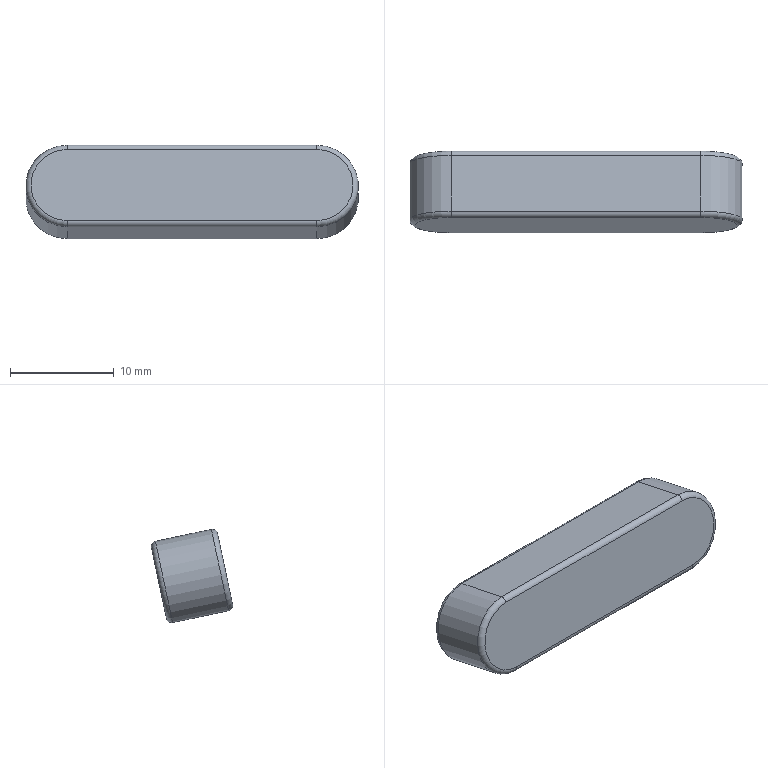Component | SolidWorks | 28ParallelKey8X32-1 | 1 solid | 14 faces | box 32 x 7.84 x 8.99 mm | volume 1567 mm3 | cylinder 6 | plane 4 | torus 4 | commonest cylinder face diameters 1 x4 8 x2
build123d program:
from build123d import *

# Parameters (mm, degrees)
BOSS_EXTRUDE1_DEPTH = 6.5
FILLET1_R           = 0.5


with BuildPart() as part:
    # Sketch1 → Boss-Extrude1 (new body)
    with BuildSketch(Plane(origin=(0, 0, 0), x_dir=(1, 0, 0), z_dir=(0, 1, 0))):
        with BuildLine():
            Line((-12, 4), (12, 4))
            ThreePointArc((12, 4), (16, 0), (12, -4))
            Line((12, -4), (-12, -4))
            ThreePointArc((-12, -4), (-16, 0), (-12, 4))
        make_face()
    extrude(amount=BOSS_EXTRUDE1_DEPTH)

    # Fillet1
    fillet1_edges = [part.edges().sort_by_distance(p)[0] for p in [
        (16, 6.5, 0),
        (0, 6.5, -4),
        (-16, 6.5, 0),
        (0, 0, -4),
        (16, 0, 0),
        (0, 0, 4),
        (-16, 0, 0),
        (0, 6.5, 4),
    ]]
    fillet(fillet1_edges, radius=FILLET1_R)


solid = part.part

# Placed as in the assembly
solid = solid.moved(Location((22.957, -20.232, 254.678), (168, 0, 0)))
STEP:
#1=COLOUR_RGB('',0.7922,0.8196,0.9333);
#2=FILL_AREA_STYLE_COLOUR('',#1);
#3=FILL_AREA_STYLE('',(#2));
#4=SURFACE_STYLE_FILL_AREA(#3);
#5=SURFACE_SIDE_STYLE('',(#4));
#6=SURFACE_STYLE_USAGE(.BOTH.,#5);
#7=PRESENTATION_STYLE_ASSIGNMENT((#6));
#8=CARTESIAN_POINT('',(0.4314,-0.8485,9.877));
#9=VERTEX_POINT('',#8);
#10=CARTESIAN_POINT('',(0.4314,-1.06,9.922));
#11=VERTEX_POINT('',#10);
#12=CARTESIAN_POINT('',(0.4314,-0.8293,9.873));
#13=DIRECTION('',(-0.,-0.9781,0.2079));
#14=VECTOR('',#13,39.37);
#15=LINE('',#12,#14);
#16=EDGE_CURVE('',#9,#11,#15,.T.);
#17=ORIENTED_EDGE('',*,*,#16,.T.);
#18=CARTESIAN_POINT('',(0.4314,-0.9949,10.23));
#19=VERTEX_POINT('',#18);
#20=CARTESIAN_POINT('',(0.4314,-1.028,10.076));
#21=DIRECTION('',(0.,0.9781,-0.2079));
#22=DIRECTION('',(0.,0.2079,0.9781));
#23=AXIS2_PLACEMENT_3D('',#20,#21,#22);
#24=CIRCLE('',#23,0.1575);
#25=EDGE_CURVE('',#11,#19,#24,.T.);
#26=ORIENTED_EDGE('',*,*,#25,.T.);
#27=CARTESIAN_POINT('',(0.4314,-0.7831,10.185));
#28=VERTEX_POINT('',#27);
#29=CARTESIAN_POINT('',(0.4314,-0.7638,10.181));
#30=DIRECTION('',(-0.,-0.9781,0.2079));
#31=VECTOR('',#30,39.37);
#32=LINE('',#29,#31);
#33=EDGE_CURVE('',#28,#19,#32,.T.);
#34=ORIENTED_EDGE('',*,*,#33,.F.);
#35=CARTESIAN_POINT('',(0.4314,-0.8158,10.031));
#36=DIRECTION('',(-0.,-0.9781,0.2079));
#37=DIRECTION('',(0.,0.2079,0.9781));
#38=AXIS2_PLACEMENT_3D('',#35,#36,#37);
#39=CIRCLE('',#38,0.1575);
#40=EDGE_CURVE('',#28,#9,#39,.T.);
#41=ORIENTED_EDGE('',*,*,#40,.T.);
#42=EDGE_LOOP('',(#17,#26,#34,#41));
#43=FACE_OUTER_BOUND('',#42,.T.);
#44=CARTESIAN_POINT('',(0.4314,-0.7965,10.027));
#45=DIRECTION('',(-0.,-0.9781,0.2079));
#46=DIRECTION('',(0.,-0.2079,-0.9781));
#47=AXIS2_PLACEMENT_3D('',#44,#45,#46);
#48=CYLINDRICAL_SURFACE('',#47,0.1575);
#49=ADVANCED_FACE('',(#43),#48,.T.);
#50=ORIENTED_EDGE('',*,*,#33,.T.);
#51=CARTESIAN_POINT('',(1.376,-0.9949,10.23));
#52=VERTEX_POINT('',#51);
#53=CARTESIAN_POINT('',(0.4314,-0.9949,10.23));
#54=DIRECTION('',(1.,-0.,0.));
#55=VECTOR('',#54,39.37);
#56=LINE('',#53,#55);
#57=EDGE_CURVE('',#19,#52,#56,.T.);
#58=ORIENTED_EDGE('',*,*,#57,.T.);
#59=CARTESIAN_POINT('',(1.376,-0.7831,10.185));
#60=VERTEX_POINT('',#59);
#61=CARTESIAN_POINT('',(1.376,-0.7638,10.181));
#62=DIRECTION('',(-0.,-0.9781,0.2079));
#63=VECTOR('',#62,39.37);
#64=LINE('',#61,#63);
#65=EDGE_CURVE('',#60,#52,#64,.T.);
#66=ORIENTED_EDGE('',*,*,#65,.F.);
#67=CARTESIAN_POINT('',(0.4314,-0.7831,10.185));
#68=DIRECTION('',(-1.,0.,-0.));
#69=VECTOR('',#68,39.37);
#70=LINE('',#67,#69);
#71=EDGE_CURVE('',#60,#28,#70,.T.);
#72=ORIENTED_EDGE('',*,*,#71,.T.);
#73=EDGE_LOOP('',(#50,#58,#66,#72));
#74=FACE_OUTER_BOUND('',#73,.T.);
#75=CARTESIAN_POINT('',(0.4314,-0.7638,10.181));
#76=DIRECTION('',(0.,-0.2079,-0.9781));
#77=DIRECTION('',(-1.,0.,-0.));
#78=AXIS2_PLACEMENT_3D('',#75,#76,#77);
#79=PLANE('',#78);
#80=ADVANCED_FACE('',(#74),#79,.F.);
#81=ORIENTED_EDGE('',*,*,#65,.T.);
#82=CARTESIAN_POINT('',(1.376,-1.06,9.922));
#83=VERTEX_POINT('',#82);
#84=CARTESIAN_POINT('',(1.376,-1.028,10.076));
#85=DIRECTION('',(0.,0.9781,-0.2079));
#86=DIRECTION('',(0.,0.2079,0.9781));
#87=AXIS2_PLACEMENT_3D('',#84,#85,#86);
#88=CIRCLE('',#87,0.1575);
#89=EDGE_CURVE('',#52,#83,#88,.T.);
#90=ORIENTED_EDGE('',*,*,#89,.T.);
#91=CARTESIAN_POINT('',(1.376,-0.8485,9.877));
#92=VERTEX_POINT('',#91);
#93=CARTESIAN_POINT('',(1.376,-0.8293,9.873));
#94=DIRECTION('',(-0.,-0.9781,0.2079));
#95=VECTOR('',#94,39.37);
#96=LINE('',#93,#95);
#97=EDGE_CURVE('',#92,#83,#96,.T.);
#98=ORIENTED_EDGE('',*,*,#97,.F.);
#99=CARTESIAN_POINT('',(1.376,-0.8158,10.031));
#100=DIRECTION('',(-0.,-0.9781,0.2079));
#101=DIRECTION('',(0.,0.2079,0.9781));
#102=AXIS2_PLACEMENT_3D('',#99,#100,#101);
#103=CIRCLE('',#102,0.1575);
#104=EDGE_CURVE('',#92,#60,#103,.T.);
#105=ORIENTED_EDGE('',*,*,#104,.T.);
#106=EDGE_LOOP('',(#81,#90,#98,#105));
#107=FACE_OUTER_BOUND('',#106,.T.);
#108=CARTESIAN_POINT('',(1.376,-0.7965,10.027));
#109=DIRECTION('',(-0.,-0.9781,0.2079));
#110=DIRECTION('',(0.,-0.2079,-0.9781));
#111=AXIS2_PLACEMENT_3D('',#108,#109,#110);
#112=CYLINDRICAL_SURFACE('',#111,0.1575);
#113=ADVANCED_FACE('',(#107),#112,.T.);
#114=ORIENTED_EDGE('',*,*,#97,.T.);
#115=CARTESIAN_POINT('',(0.4314,-1.06,9.922));
#116=DIRECTION('',(-1.,0.,-0.));
#117=VECTOR('',#116,39.37);
#118=LINE('',#115,#117);
#119=EDGE_CURVE('',#83,#11,#118,.T.);
#120=ORIENTED_EDGE('',*,*,#119,.T.);
#121=ORIENTED_EDGE('',*,*,#16,.F.);
#122=CARTESIAN_POINT('',(1.376,-0.8485,9.877));
#123=DIRECTION('',(1.,-0.,0.));
#124=VECTOR('',#123,39.37);
#125=LINE('',#122,#124);
#126=EDGE_CURVE('',#9,#92,#125,.T.);
#127=ORIENTED_EDGE('',*,*,#126,.T.);
#128=EDGE_LOOP('',(#114,#120,#121,#127));
#129=FACE_OUTER_BOUND('',#128,.T.);
#130=CARTESIAN_POINT('',(0.4314,-0.8293,9.873));
#131=DIRECTION('',(-0.,0.2079,0.9781));
#132=DIRECTION('',(1.,-0.,0.));
#133=AXIS2_PLACEMENT_3D('',#130,#131,#132);
#134=PLANE('',#133);
#135=ADVANCED_FACE('',(#129),#134,.F.);
#136=CARTESIAN_POINT('',(1.376,-0.7679,10.161));
#137=VERTEX_POINT('',#136);
#138=CARTESIAN_POINT('',(1.376,-0.8252,9.892));
#139=VERTEX_POINT('',#138);
#140=CARTESIAN_POINT('',(1.376,-0.7965,10.027));
#141=DIRECTION('',(0.,0.9781,-0.2079));
#142=DIRECTION('',(0.,0.2079,0.9781));
#143=AXIS2_PLACEMENT_3D('',#140,#141,#142);
#144=CIRCLE('',#143,0.1378);
#145=EDGE_CURVE('',#137,#139,#144,.T.);
#146=ORIENTED_EDGE('',*,*,#145,.T.);
#147=CARTESIAN_POINT('',(0.4314,-0.8252,9.892));
#148=VERTEX_POINT('',#147);
#149=CARTESIAN_POINT('',(0.4314,-0.8252,9.892));
#150=DIRECTION('',(-1.,0.,-0.));
#151=VECTOR('',#150,39.37);
#152=LINE('',#149,#151);
#153=EDGE_CURVE('',#139,#148,#152,.T.);
#154=ORIENTED_EDGE('',*,*,#153,.T.);
#155=CARTESIAN_POINT('',(0.4314,-0.7679,10.161));
#156=VERTEX_POINT('',#155);
#157=CARTESIAN_POINT('',(0.4314,-0.7965,10.027));
#158=DIRECTION('',(0.,0.9781,-0.2079));
#159=DIRECTION('',(0.,0.2079,0.9781));
#160=AXIS2_PLACEMENT_3D('',#157,#158,#159);
#161=CIRCLE('',#160,0.1378);
#162=EDGE_CURVE('',#148,#156,#161,.T.);
#163=ORIENTED_EDGE('',*,*,#162,.T.);
#164=CARTESIAN_POINT('',(1.376,-0.7679,10.161));
#165=DIRECTION('',(1.,-0.,0.));
#166=VECTOR('',#165,39.37);
#167=LINE('',#164,#166);
#168=EDGE_CURVE('',#156,#137,#167,.T.);
#169=ORIENTED_EDGE('',*,*,#168,.T.);
#170=EDGE_LOOP('',(#146,#154,#163,#169));
#171=FACE_OUTER_BOUND('',#170,.T.);
#172=CARTESIAN_POINT('',(0.4314,-0.7965,10.027));
#173=DIRECTION('',(0.,0.9781,-0.2079));
#174=DIRECTION('',(-0.,0.2079,0.9781));
#175=AXIS2_PLACEMENT_3D('',#172,#173,#174);
#176=PLANE('',#175);
#177=ADVANCED_FACE('',(#171),#176,.T.);
#178=CARTESIAN_POINT('',(1.376,-1.076,9.945));
#179=VERTEX_POINT('',#178);
#180=CARTESIAN_POINT('',(1.376,-1.018,10.215));
#181=VERTEX_POINT('',#180);
#182=CARTESIAN_POINT('',(1.376,-1.047,10.08));
#183=DIRECTION('',(-0.,-0.9781,0.2079));
#184=DIRECTION('',(0.,0.2079,0.9781));
#185=AXIS2_PLACEMENT_3D('',#182,#183,#184);
#186=CIRCLE('',#185,0.1378);
#187=EDGE_CURVE('',#179,#181,#186,.T.);
#188=ORIENTED_EDGE('',*,*,#187,.T.);
#189=CARTESIAN_POINT('',(0.4314,-1.018,10.215));
#190=VERTEX_POINT('',#189);
#191=CARTESIAN_POINT('',(0.4314,-1.018,10.215));
#192=DIRECTION('',(-1.,0.,-0.));
#193=VECTOR('',#192,39.37);
#194=LINE('',#191,#193);
#195=EDGE_CURVE('',#181,#190,#194,.T.);
#196=ORIENTED_EDGE('',*,*,#195,.T.);
#197=CARTESIAN_POINT('',(0.4314,-1.076,9.945));
#198=VERTEX_POINT('',#197);
#199=CARTESIAN_POINT('',(0.4314,-1.047,10.08));
#200=DIRECTION('',(-0.,-0.9781,0.2079));
#201=DIRECTION('',(0.,0.2079,0.9781));
#202=AXIS2_PLACEMENT_3D('',#199,#200,#201);
#203=CIRCLE('',#202,0.1378);
#204=EDGE_CURVE('',#190,#198,#203,.T.);
#205=ORIENTED_EDGE('',*,*,#204,.T.);
#206=CARTESIAN_POINT('',(0.4314,-1.076,9.945));
#207=DIRECTION('',(1.,-0.,0.));
#208=VECTOR('',#207,39.37);
#209=LINE('',#206,#208);
#210=EDGE_CURVE('',#198,#179,#209,.T.);
#211=ORIENTED_EDGE('',*,*,#210,.T.);
#212=EDGE_LOOP('',(#188,#196,#205,#211));
#213=FACE_OUTER_BOUND('',#212,.T.);
#214=CARTESIAN_POINT('',(0.4314,-1.047,10.08));
#215=DIRECTION('',(0.,0.9781,-0.2079));
#216=DIRECTION('',(-0.,0.2079,0.9781));
#217=AXIS2_PLACEMENT_3D('',#214,#215,#216);
#218=PLANE('',#217);
#219=ADVANCED_FACE('',(#213),#218,.F.);
#220=CARTESIAN_POINT('',(1.376,-1.056,9.941));
#221=DIRECTION('',(1.,-0.,0.));
#222=DIRECTION('',(0.,-0.2079,-0.9781));
#223=AXIS2_PLACEMENT_3D('',#220,#221,#222);
#224=CIRCLE('',#223,0.01969);
#225=EDGE_CURVE('',#179,#83,#224,.T.);
#226=ORIENTED_EDGE('',*,*,#225,.F.);
#227=ORIENTED_EDGE('',*,*,#210,.F.);
#228=CARTESIAN_POINT('',(0.4314,-1.056,9.941));
#229=DIRECTION('',(-1.,0.,-0.));
#230=DIRECTION('',(0.,0.2079,0.9781));
#231=AXIS2_PLACEMENT_3D('',#228,#229,#230);
#232=CIRCLE('',#231,0.01969);
#233=EDGE_CURVE('',#11,#198,#232,.T.);
#234=ORIENTED_EDGE('',*,*,#233,.F.);
#235=ORIENTED_EDGE('',*,*,#119,.F.);
#236=EDGE_LOOP('',(#226,#227,#234,#235));
#237=FACE_OUTER_BOUND('',#236,.T.);
#238=CARTESIAN_POINT('',(0.4314,-1.056,9.941));
#239=DIRECTION('',(-1.,0.,-0.));
#240=DIRECTION('',(0.,0.2079,0.9781));
#241=AXIS2_PLACEMENT_3D('',#238,#239,#240);
#242=CYLINDRICAL_SURFACE('',#241,0.01969);
#243=ADVANCED_FACE('',(#237),#242,.T.);
#244=ORIENTED_EDGE('',*,*,#233,.T.);
#245=ORIENTED_EDGE('',*,*,#204,.F.);
#246=CARTESIAN_POINT('',(0.4314,-0.999,10.211));
#247=DIRECTION('',(1.,-0.,0.));
#248=DIRECTION('',(0.,-0.2079,-0.9781));
#249=AXIS2_PLACEMENT_3D('',#246,#247,#248);
#250=CIRCLE('',#249,0.01969);
#251=EDGE_CURVE('',#19,#190,#250,.T.);
#252=ORIENTED_EDGE('',*,*,#251,.F.);
#253=ORIENTED_EDGE('',*,*,#25,.F.);
#254=EDGE_LOOP('',(#244,#245,#252,#253));
#255=FACE_OUTER_BOUND('',#254,.T.);
#256=CARTESIAN_POINT('',(0.4314,-1.028,10.076));
#257=DIRECTION('',(0.,0.9781,-0.2079));
#258=DIRECTION('',(0.,0.2079,0.9781));
#259=AXIS2_PLACEMENT_3D('',#256,#257,#258);
#260=TOROIDAL_SURFACE('',#259,0.1378,0.01969);
#261=ADVANCED_FACE('',(#255),#260,.T.);
#262=ORIENTED_EDGE('',*,*,#225,.T.);
#263=ORIENTED_EDGE('',*,*,#89,.F.);
#264=CARTESIAN_POINT('',(1.376,-0.999,10.211));
#265=DIRECTION('',(-1.,0.,-0.));
#266=DIRECTION('',(0.,0.2079,0.9781));
#267=AXIS2_PLACEMENT_3D('',#264,#265,#266);
#268=CIRCLE('',#267,0.01969);
#269=EDGE_CURVE('',#181,#52,#268,.T.);
#270=ORIENTED_EDGE('',*,*,#269,.F.);
#271=ORIENTED_EDGE('',*,*,#187,.F.);
#272=EDGE_LOOP('',(#262,#263,#270,#271));
#273=FACE_OUTER_BOUND('',#272,.T.);
#274=CARTESIAN_POINT('',(1.376,-1.028,10.076));
#275=DIRECTION('',(0.,0.9781,-0.2079));
#276=DIRECTION('',(0.,0.2079,0.9781));
#277=AXIS2_PLACEMENT_3D('',#274,#275,#276);
#278=TOROIDAL_SURFACE('',#277,0.1378,0.01969);
#279=ADVANCED_FACE('',(#273),#278,.T.);
#280=ORIENTED_EDGE('',*,*,#251,.T.);
#281=ORIENTED_EDGE('',*,*,#195,.F.);
#282=ORIENTED_EDGE('',*,*,#269,.T.);
#283=ORIENTED_EDGE('',*,*,#57,.F.);
#284=EDGE_LOOP('',(#280,#281,#282,#283));
#285=FACE_OUTER_BOUND('',#284,.T.);
#286=CARTESIAN_POINT('',(0.4314,-0.999,10.211));
#287=DIRECTION('',(1.,-0.,0.));
#288=DIRECTION('',(0.,-0.2079,-0.9781));
#289=AXIS2_PLACEMENT_3D('',#286,#287,#288);
#290=CYLINDRICAL_SURFACE('',#289,0.01969);
#291=ADVANCED_FACE('',(#285),#290,.T.);
#292=CARTESIAN_POINT('',(0.4314,-0.7872,10.166));
#293=DIRECTION('',(-1.,0.,-0.));
#294=DIRECTION('',(0.,0.2079,0.9781));
#295=AXIS2_PLACEMENT_3D('',#292,#293,#294);
#296=CIRCLE('',#295,0.01969);
#297=EDGE_CURVE('',#28,#156,#296,.T.);
#298=ORIENTED_EDGE('',*,*,#297,.F.);
#299=ORIENTED_EDGE('',*,*,#71,.F.);
#300=CARTESIAN_POINT('',(1.376,-0.7872,10.166));
#301=DIRECTION('',(1.,-0.,0.));
#302=DIRECTION('',(0.,-0.2079,-0.9781));
#303=AXIS2_PLACEMENT_3D('',#300,#301,#302);
#304=CIRCLE('',#303,0.01969);
#305=EDGE_CURVE('',#137,#60,#304,.T.);
#306=ORIENTED_EDGE('',*,*,#305,.F.);
#307=ORIENTED_EDGE('',*,*,#168,.F.);
#308=EDGE_LOOP('',(#298,#299,#306,#307));
#309=FACE_OUTER_BOUND('',#308,.T.);
#310=CARTESIAN_POINT('',(0.4314,-0.7872,10.166));
#311=DIRECTION('',(-1.,0.,-0.));
#312=DIRECTION('',(0.,0.2079,0.9781));
#313=AXIS2_PLACEMENT_3D('',#310,#311,#312);
#314=CYLINDRICAL_SURFACE('',#313,0.01969);
#315=ADVANCED_FACE('',(#309),#314,.T.);
#316=ORIENTED_EDGE('',*,*,#305,.T.);
#317=ORIENTED_EDGE('',*,*,#104,.F.);
#318=CARTESIAN_POINT('',(1.376,-0.8445,9.896));
#319=DIRECTION('',(-1.,0.,-0.));
#320=DIRECTION('',(0.,0.2079,0.9781));
#321=AXIS2_PLACEMENT_3D('',#318,#319,#320);
#322=CIRCLE('',#321,0.01969);
#323=EDGE_CURVE('',#139,#92,#322,.T.);
#324=ORIENTED_EDGE('',*,*,#323,.F.);
#325=ORIENTED_EDGE('',*,*,#145,.F.);
#326=EDGE_LOOP('',(#316,#317,#324,#325));
#327=FACE_OUTER_BOUND('',#326,.T.);
#328=CARTESIAN_POINT('',(1.376,-0.8158,10.031));
#329=DIRECTION('',(0.,0.9781,-0.2079));
#330=DIRECTION('',(0.,0.2079,0.9781));
#331=AXIS2_PLACEMENT_3D('',#328,#329,#330);
#332=TOROIDAL_SURFACE('',#331,0.1378,0.01969);
#333=ADVANCED_FACE('',(#327),#332,.T.);
#334=ORIENTED_EDGE('',*,*,#297,.T.);
#335=ORIENTED_EDGE('',*,*,#162,.F.);
#336=CARTESIAN_POINT('',(0.4314,-0.8445,9.896));
#337=DIRECTION('',(1.,-0.,0.));
#338=DIRECTION('',(0.,-0.2079,-0.9781));
#339=AXIS2_PLACEMENT_3D('',#336,#337,#338);
#340=CIRCLE('',#339,0.01969);
#341=EDGE_CURVE('',#9,#148,#340,.T.);
#342=ORIENTED_EDGE('',*,*,#341,.F.);
#343=ORIENTED_EDGE('',*,*,#40,.F.);
#344=EDGE_LOOP('',(#334,#335,#342,#343));
#345=FACE_OUTER_BOUND('',#344,.T.);
#346=CARTESIAN_POINT('',(0.4314,-0.8158,10.031));
#347=DIRECTION('',(0.,0.9781,-0.2079));
#348=DIRECTION('',(0.,0.2079,0.9781));
#349=AXIS2_PLACEMENT_3D('',#346,#347,#348);
#350=TOROIDAL_SURFACE('',#349,0.1378,0.01969);
#351=ADVANCED_FACE('',(#345),#350,.T.);
#352=ORIENTED_EDGE('',*,*,#323,.T.);
#353=ORIENTED_EDGE('',*,*,#126,.F.);
#354=ORIENTED_EDGE('',*,*,#341,.T.);
#355=ORIENTED_EDGE('',*,*,#153,.F.);
#356=EDGE_LOOP('',(#352,#353,#354,#355));
#357=FACE_OUTER_BOUND('',#356,.T.);
#358=CARTESIAN_POINT('',(0.4314,-0.8445,9.896));
#359=DIRECTION('',(1.,-0.,0.));
#360=DIRECTION('',(0.,-0.2079,-0.9781));
#361=AXIS2_PLACEMENT_3D('',#358,#359,#360);
#362=CYLINDRICAL_SURFACE('',#361,0.01969);
#363=ADVANCED_FACE('',(#357),#362,.T.);
#364=CLOSED_SHELL('',(#49,#80,#113,#135,#177,#219,#243,#261,#279,#291,#315,#333,#351,#363));
#365=MANIFOLD_SOLID_BREP('',#364);
#366=STYLED_ITEM('',(#7),#365);
#367=(LENGTH_UNIT()NAMED_UNIT(*)SI_UNIT($,.METRE.));
#368=LENGTH_MEASURE_WITH_UNIT(LENGTH_MEASURE(0.0254),#367);
#369=DIMENSIONAL_EXPONENTS(1.,0.,0.,0.,0.,0.,0.);
#370=(CONVERSION_BASED_UNIT('',#368)LENGTH_UNIT()NAMED_UNIT(#369));
#371=UNCERTAINTY_MEASURE_WITH_UNIT(LENGTH_MEASURE(0.00001),#370,'','');
#372=(NAMED_UNIT(*)PLANE_ANGLE_UNIT()SI_UNIT($,.RADIAN.));
#373=(NAMED_UNIT(*)SI_UNIT($,.STERADIAN.)SOLID_ANGLE_UNIT());
#374=(GEOMETRIC_REPRESENTATION_CONTEXT(3)GLOBAL_UNCERTAINTY_ASSIGNED_CONTEXT((#371))GLOBAL_UNIT_ASSIGNED_CONTEXT((#370,#372,#373))REPRESENTATION_CONTEXT('',''));
#375=MECHANICAL_DESIGN_GEOMETRIC_PRESENTATION_REPRESENTATION('',(#366),#374);
#376=PRESENTATION_LAYER_ASSIGNMENT('','',(#366));
#377=CARTESIAN_POINT('',(0.,0.,0.));
#378=DIRECTION('',(0.,0.,1.));
#379=DIRECTION('',(1.,0.,0.));
#380=AXIS2_PLACEMENT_3D('',#377,#378,#379);
#381=(LENGTH_UNIT()NAMED_UNIT(*)SI_UNIT($,.METRE.));
#382=LENGTH_MEASURE_WITH_UNIT(LENGTH_MEASURE(0.0254),#381);
#383=DIMENSIONAL_EXPONENTS(1.,0.,0.,0.,0.,0.,0.);
#384=(CONVERSION_BASED_UNIT('',#382)LENGTH_UNIT()NAMED_UNIT(#383));
#385=UNCERTAINTY_MEASURE_WITH_UNIT(LENGTH_MEASURE(0.00001),#384,'','');
#386=(NAMED_UNIT(*)PLANE_ANGLE_UNIT()SI_UNIT($,.RADIAN.));
#387=(NAMED_UNIT(*)SI_UNIT($,.STERADIAN.)SOLID_ANGLE_UNIT());
#388=(GEOMETRIC_REPRESENTATION_CONTEXT(3)GLOBAL_UNCERTAINTY_ASSIGNED_CONTEXT((#385))GLOBAL_UNIT_ASSIGNED_CONTEXT((#384,#386,#387))REPRESENTATION_CONTEXT('',''));
#389=ADVANCED_BREP_SHAPE_REPRESENTATION('',(#365,#380),#388);